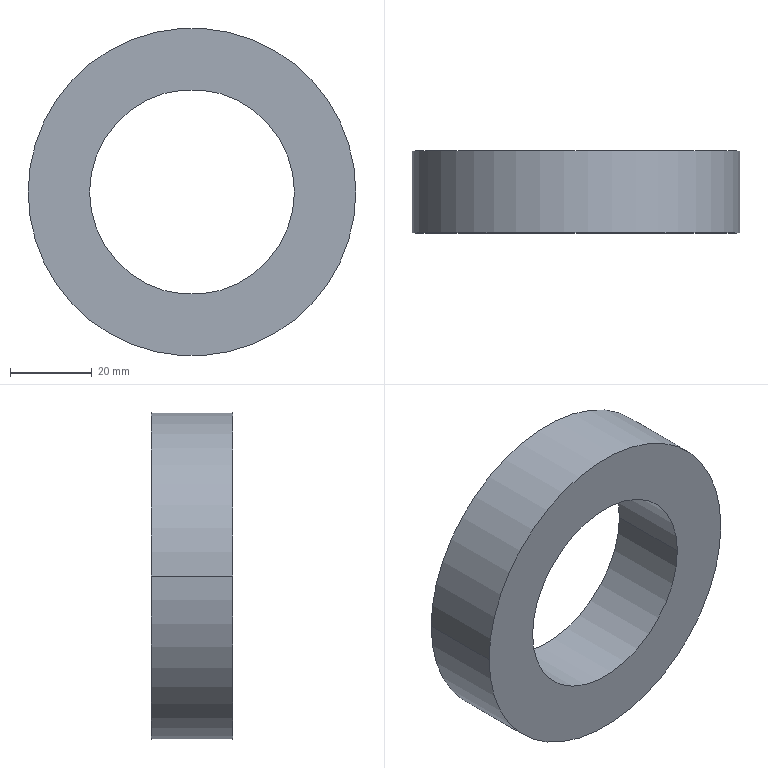Component | SolidWorks | RetainingRing-2 | 1 solid | 6 faces | box 80 x 20 x 80 mm | volume 61261 mm3 | cylinder 4 | plane 2 | commonest cylinder face diameters 50 x2 80 x2
build123d program:
from build123d import *

# Parameters (mm, degrees)
SKETCH1_R           = 40
SKETCH1_R_2         = 25
BOSS_EXTRUDE1_DEPTH = 20


with BuildPart() as part:
    # Sketch1 → Boss-Extrude1 (new body)
    with BuildSketch(Plane.XY):
        with Locations((-327.615, 384.486)):
            Circle(SKETCH1_R)
        with Locations((-327.615, 384.486)):
            Circle(SKETCH1_R_2, mode=Mode.SUBTRACT)
    extrude(amount=BOSS_EXTRUDE1_DEPTH)


solid = part.part

# Placed as in the assembly
solid = solid.moved(Location((8.644, -741, -723.781), (90, 0, 0)))
STEP:
#1=COLOUR_RGB('',0.7922,0.8196,0.9333);
#2=FILL_AREA_STYLE_COLOUR('',#1);
#3=FILL_AREA_STYLE('',(#2));
#4=SURFACE_STYLE_FILL_AREA(#3);
#5=SURFACE_SIDE_STYLE('',(#4));
#6=SURFACE_STYLE_USAGE(.BOTH.,#5);
#7=PRESENTATION_STYLE_ASSIGNMENT((#6));
#8=CARTESIAN_POINT('',(-13.542,-29.173,-13.358));
#9=VERTEX_POINT('',#8);
#10=CARTESIAN_POINT('',(-11.574,-29.173,-13.358));
#11=VERTEX_POINT('',#10);
#12=CARTESIAN_POINT('',(-12.558,-29.173,-13.358));
#13=DIRECTION('',(-0.,1.,0.));
#14=DIRECTION('',(1.,0.,0.));
#15=AXIS2_PLACEMENT_3D('',#12,#13,#14);
#16=CIRCLE('',#15,0.9843);
#17=EDGE_CURVE('',#9,#11,#16,.T.);
#18=ORIENTED_EDGE('',*,*,#17,.T.);
#19=CARTESIAN_POINT('',(-11.574,-29.961,-13.358));
#20=VERTEX_POINT('',#19);
#21=CARTESIAN_POINT('',(-11.574,-29.173,-13.358));
#22=DIRECTION('',(0.,-1.,-0.));
#23=VECTOR('',#22,39.37);
#24=LINE('',#21,#23);
#25=EDGE_CURVE('',#11,#20,#24,.T.);
#26=ORIENTED_EDGE('',*,*,#25,.T.);
#27=CARTESIAN_POINT('',(-13.542,-29.961,-13.358));
#28=VERTEX_POINT('',#27);
#29=CARTESIAN_POINT('',(-12.558,-29.961,-13.358));
#30=DIRECTION('',(-0.,1.,0.));
#31=DIRECTION('',(1.,0.,0.));
#32=AXIS2_PLACEMENT_3D('',#29,#30,#31);
#33=CIRCLE('',#32,0.9843);
#34=EDGE_CURVE('',#28,#20,#33,.T.);
#35=ORIENTED_EDGE('',*,*,#34,.F.);
#36=CARTESIAN_POINT('',(-13.542,-29.173,-13.358));
#37=DIRECTION('',(0.,-1.,-0.));
#38=VECTOR('',#37,39.37);
#39=LINE('',#36,#38);
#40=EDGE_CURVE('',#9,#28,#39,.T.);
#41=ORIENTED_EDGE('',*,*,#40,.F.);
#42=EDGE_LOOP('',(#18,#26,#35,#41));
#43=FACE_OUTER_BOUND('',#42,.T.);
#44=CARTESIAN_POINT('',(-12.558,-29.173,-13.358));
#45=DIRECTION('',(0.,-1.,-0.));
#46=DIRECTION('',(-1.,0.,0.));
#47=AXIS2_PLACEMENT_3D('',#44,#45,#46);
#48=CYLINDRICAL_SURFACE('',#47,0.9843);
#49=ADVANCED_FACE('',(#43),#48,.F.);
#50=CARTESIAN_POINT('',(-10.983,-29.173,-13.358));
#51=VERTEX_POINT('',#50);
#52=CARTESIAN_POINT('',(-14.133,-29.173,-13.358));
#53=VERTEX_POINT('',#52);
#54=CARTESIAN_POINT('',(-12.558,-29.173,-13.358));
#55=DIRECTION('',(-0.,1.,0.));
#56=DIRECTION('',(1.,0.,0.));
#57=AXIS2_PLACEMENT_3D('',#54,#55,#56);
#58=CIRCLE('',#57,1.575);
#59=EDGE_CURVE('',#51,#53,#58,.T.);
#60=ORIENTED_EDGE('',*,*,#59,.F.);
#61=CARTESIAN_POINT('',(-10.983,-29.961,-13.358));
#62=VERTEX_POINT('',#61);
#63=CARTESIAN_POINT('',(-10.983,-29.173,-13.358));
#64=DIRECTION('',(0.,-1.,-0.));
#65=VECTOR('',#64,39.37);
#66=LINE('',#63,#65);
#67=EDGE_CURVE('',#51,#62,#66,.T.);
#68=ORIENTED_EDGE('',*,*,#67,.T.);
#69=CARTESIAN_POINT('',(-14.133,-29.961,-13.358));
#70=VERTEX_POINT('',#69);
#71=CARTESIAN_POINT('',(-12.558,-29.961,-13.358));
#72=DIRECTION('',(-0.,1.,0.));
#73=DIRECTION('',(1.,0.,0.));
#74=AXIS2_PLACEMENT_3D('',#71,#72,#73);
#75=CIRCLE('',#74,1.575);
#76=EDGE_CURVE('',#62,#70,#75,.T.);
#77=ORIENTED_EDGE('',*,*,#76,.T.);
#78=CARTESIAN_POINT('',(-14.133,-29.173,-13.358));
#79=DIRECTION('',(0.,-1.,-0.));
#80=VECTOR('',#79,39.37);
#81=LINE('',#78,#80);
#82=EDGE_CURVE('',#53,#70,#81,.T.);
#83=ORIENTED_EDGE('',*,*,#82,.F.);
#84=EDGE_LOOP('',(#60,#68,#77,#83));
#85=FACE_OUTER_BOUND('',#84,.T.);
#86=CARTESIAN_POINT('',(-12.558,-29.173,-13.358));
#87=DIRECTION('',(0.,-1.,-0.));
#88=DIRECTION('',(-1.,0.,0.));
#89=AXIS2_PLACEMENT_3D('',#86,#87,#88);
#90=CYLINDRICAL_SURFACE('',#89,1.575);
#91=ADVANCED_FACE('',(#85),#90,.T.);
#92=CARTESIAN_POINT('',(-12.558,-29.173,-13.358));
#93=DIRECTION('',(-0.,1.,0.));
#94=DIRECTION('',(1.,0.,0.));
#95=AXIS2_PLACEMENT_3D('',#92,#93,#94);
#96=CIRCLE('',#95,1.575);
#97=EDGE_CURVE('',#53,#51,#96,.T.);
#98=ORIENTED_EDGE('',*,*,#97,.T.);
#99=ORIENTED_EDGE('',*,*,#59,.T.);
#100=EDGE_LOOP('',(#98,#99));
#101=FACE_OUTER_BOUND('',#100,.T.);
#102=ORIENTED_EDGE('',*,*,#17,.F.);
#103=CARTESIAN_POINT('',(-12.558,-29.173,-13.358));
#104=DIRECTION('',(-0.,1.,0.));
#105=DIRECTION('',(1.,0.,0.));
#106=AXIS2_PLACEMENT_3D('',#103,#104,#105);
#107=CIRCLE('',#106,0.9843);
#108=EDGE_CURVE('',#11,#9,#107,.T.);
#109=ORIENTED_EDGE('',*,*,#108,.F.);
#110=EDGE_LOOP('',(#102,#109));
#111=FACE_BOUND('',#110,.T.);
#112=CARTESIAN_POINT('',(-12.558,-29.173,-13.358));
#113=DIRECTION('',(-0.,1.,0.));
#114=DIRECTION('',(1.,0.,0.));
#115=AXIS2_PLACEMENT_3D('',#112,#113,#114);
#116=PLANE('',#115);
#117=ADVANCED_FACE('',(#101,#111),#116,.T.);
#118=CARTESIAN_POINT('',(-12.558,-29.961,-13.358));
#119=DIRECTION('',(-0.,1.,0.));
#120=DIRECTION('',(1.,0.,0.));
#121=AXIS2_PLACEMENT_3D('',#118,#119,#120);
#122=CIRCLE('',#121,1.575);
#123=EDGE_CURVE('',#70,#62,#122,.T.);
#124=ORIENTED_EDGE('',*,*,#123,.F.);
#125=ORIENTED_EDGE('',*,*,#76,.F.);
#126=EDGE_LOOP('',(#124,#125));
#127=FACE_OUTER_BOUND('',#126,.T.);
#128=ORIENTED_EDGE('',*,*,#34,.T.);
#129=CARTESIAN_POINT('',(-12.558,-29.961,-13.358));
#130=DIRECTION('',(-0.,1.,0.));
#131=DIRECTION('',(1.,0.,0.));
#132=AXIS2_PLACEMENT_3D('',#129,#130,#131);
#133=CIRCLE('',#132,0.9843);
#134=EDGE_CURVE('',#20,#28,#133,.T.);
#135=ORIENTED_EDGE('',*,*,#134,.T.);
#136=EDGE_LOOP('',(#128,#135));
#137=FACE_BOUND('',#136,.T.);
#138=CARTESIAN_POINT('',(-12.558,-29.961,-13.358));
#139=DIRECTION('',(-0.,1.,0.));
#140=DIRECTION('',(1.,0.,0.));
#141=AXIS2_PLACEMENT_3D('',#138,#139,#140);
#142=PLANE('',#141);
#143=ADVANCED_FACE('',(#127,#137),#142,.F.);
#144=ORIENTED_EDGE('',*,*,#67,.F.);
#145=ORIENTED_EDGE('',*,*,#97,.F.);
#146=ORIENTED_EDGE('',*,*,#82,.T.);
#147=ORIENTED_EDGE('',*,*,#123,.T.);
#148=EDGE_LOOP('',(#144,#145,#146,#147));
#149=FACE_OUTER_BOUND('',#148,.T.);
#150=CARTESIAN_POINT('',(-12.558,-29.173,-13.358));
#151=DIRECTION('',(0.,-1.,-0.));
#152=DIRECTION('',(-1.,0.,0.));
#153=AXIS2_PLACEMENT_3D('',#150,#151,#152);
#154=CYLINDRICAL_SURFACE('',#153,1.575);
#155=ADVANCED_FACE('',(#149),#154,.T.);
#156=ORIENTED_EDGE('',*,*,#25,.F.);
#157=ORIENTED_EDGE('',*,*,#108,.T.);
#158=ORIENTED_EDGE('',*,*,#40,.T.);
#159=ORIENTED_EDGE('',*,*,#134,.F.);
#160=EDGE_LOOP('',(#156,#157,#158,#159));
#161=FACE_OUTER_BOUND('',#160,.T.);
#162=CARTESIAN_POINT('',(-12.558,-29.173,-13.358));
#163=DIRECTION('',(0.,-1.,-0.));
#164=DIRECTION('',(-1.,0.,0.));
#165=AXIS2_PLACEMENT_3D('',#162,#163,#164);
#166=CYLINDRICAL_SURFACE('',#165,0.9843);
#167=ADVANCED_FACE('',(#161),#166,.F.);
#168=CLOSED_SHELL('',(#49,#91,#117,#143,#155,#167));
#169=MANIFOLD_SOLID_BREP('',#168);
#170=STYLED_ITEM('',(#7),#169);
#171=PRESENTATION_LAYER_ASSIGNMENT('','',(#170));
#172=CARTESIAN_POINT('',(0.,0.,0.));
#173=DIRECTION('',(0.,0.,1.));
#174=DIRECTION('',(1.,0.,0.));
#175=AXIS2_PLACEMENT_3D('',#172,#173,#174);
#176=(LENGTH_UNIT()NAMED_UNIT(*)SI_UNIT($,.METRE.));
#177=LENGTH_MEASURE_WITH_UNIT(LENGTH_MEASURE(0.0254),#176);
#178=DIMENSIONAL_EXPONENTS(1.,0.,0.,0.,0.,0.,0.);
#179=(CONVERSION_BASED_UNIT('',#177)LENGTH_UNIT()NAMED_UNIT(#178));
#180=UNCERTAINTY_MEASURE_WITH_UNIT(LENGTH_MEASURE(0.00001),#179,'','');
#181=(NAMED_UNIT(*)PLANE_ANGLE_UNIT()SI_UNIT($,.RADIAN.));
#182=(NAMED_UNIT(*)SI_UNIT($,.STERADIAN.)SOLID_ANGLE_UNIT());
#183=(GEOMETRIC_REPRESENTATION_CONTEXT(3)GLOBAL_UNCERTAINTY_ASSIGNED_CONTEXT((#180))GLOBAL_UNIT_ASSIGNED_CONTEXT((#179,#181,#182))REPRESENTATION_CONTEXT('',''));
#184=ADVANCED_BREP_SHAPE_REPRESENTATION('',(#169,#175),#183);
#185=(LENGTH_UNIT()NAMED_UNIT(*)SI_UNIT($,.METRE.));
#186=LENGTH_MEASURE_WITH_UNIT(LENGTH_MEASURE(0.0254),#185);
#187=DIMENSIONAL_EXPONENTS(1.,0.,0.,0.,0.,0.,0.);
#188=(CONVERSION_BASED_UNIT('',#186)LENGTH_UNIT()NAMED_UNIT(#187));
#189=UNCERTAINTY_MEASURE_WITH_UNIT(LENGTH_MEASURE(0.00001),#188,'','');
#190=(NAMED_UNIT(*)PLANE_ANGLE_UNIT()SI_UNIT($,.RADIAN.));
#191=(NAMED_UNIT(*)SI_UNIT($,.STERADIAN.)SOLID_ANGLE_UNIT());
#192=(GEOMETRIC_REPRESENTATION_CONTEXT(3)GLOBAL_UNCERTAINTY_ASSIGNED_CONTEXT((#189))GLOBAL_UNIT_ASSIGNED_CONTEXT((#188,#190,#191))REPRESENTATION_CONTEXT('',''));
#193=MECHANICAL_DESIGN_GEOMETRIC_PRESENTATION_REPRESENTATION('',(#170),#192);